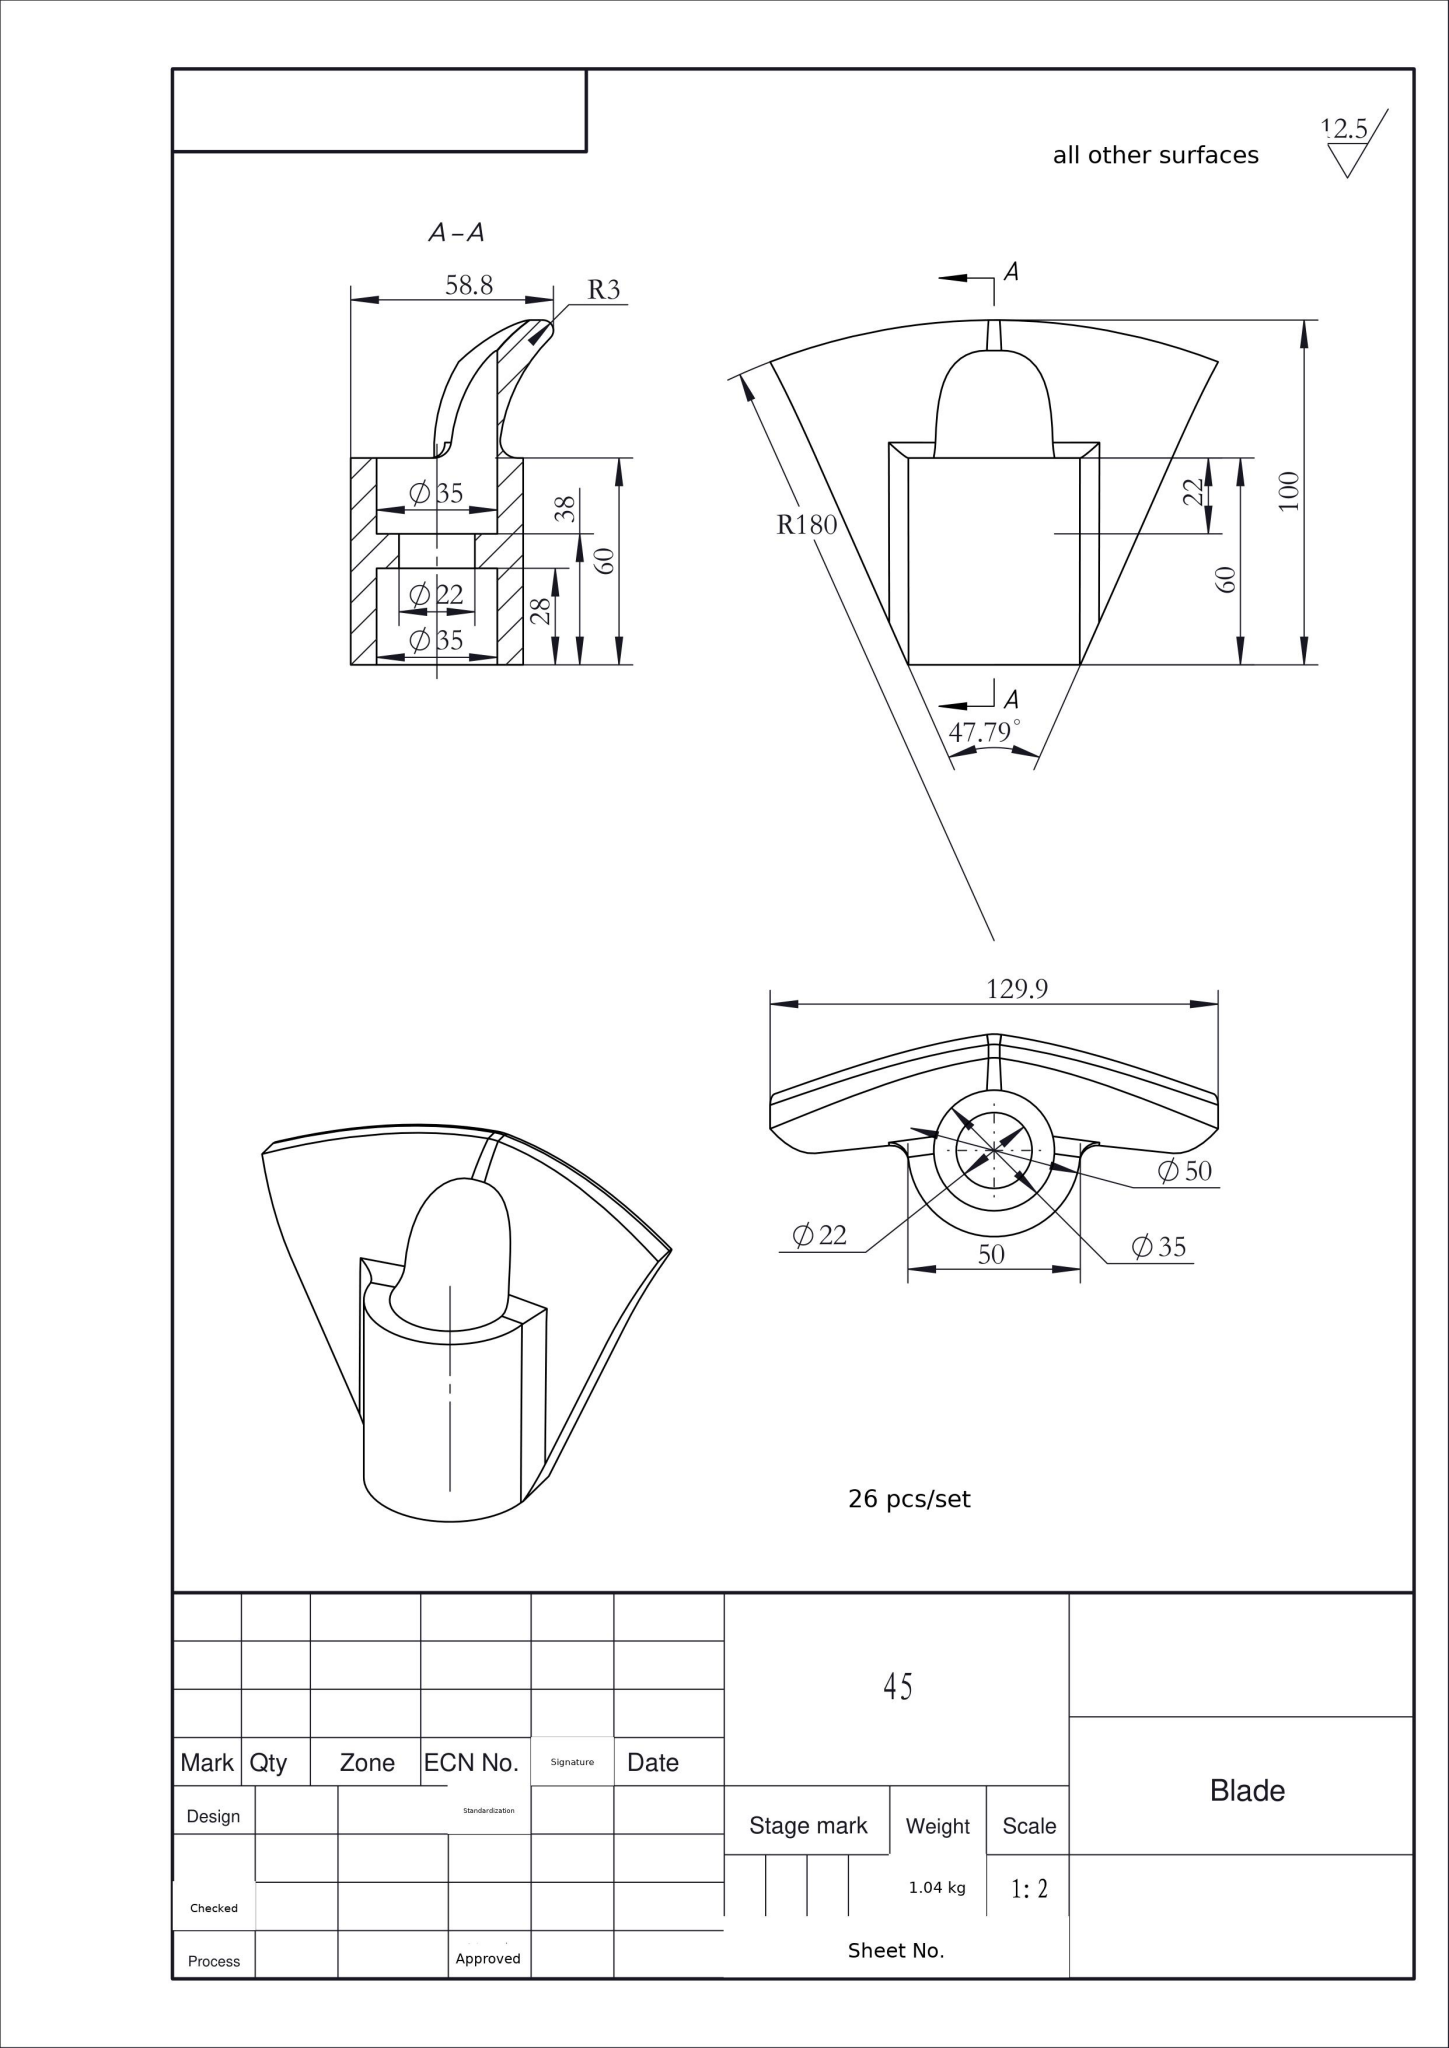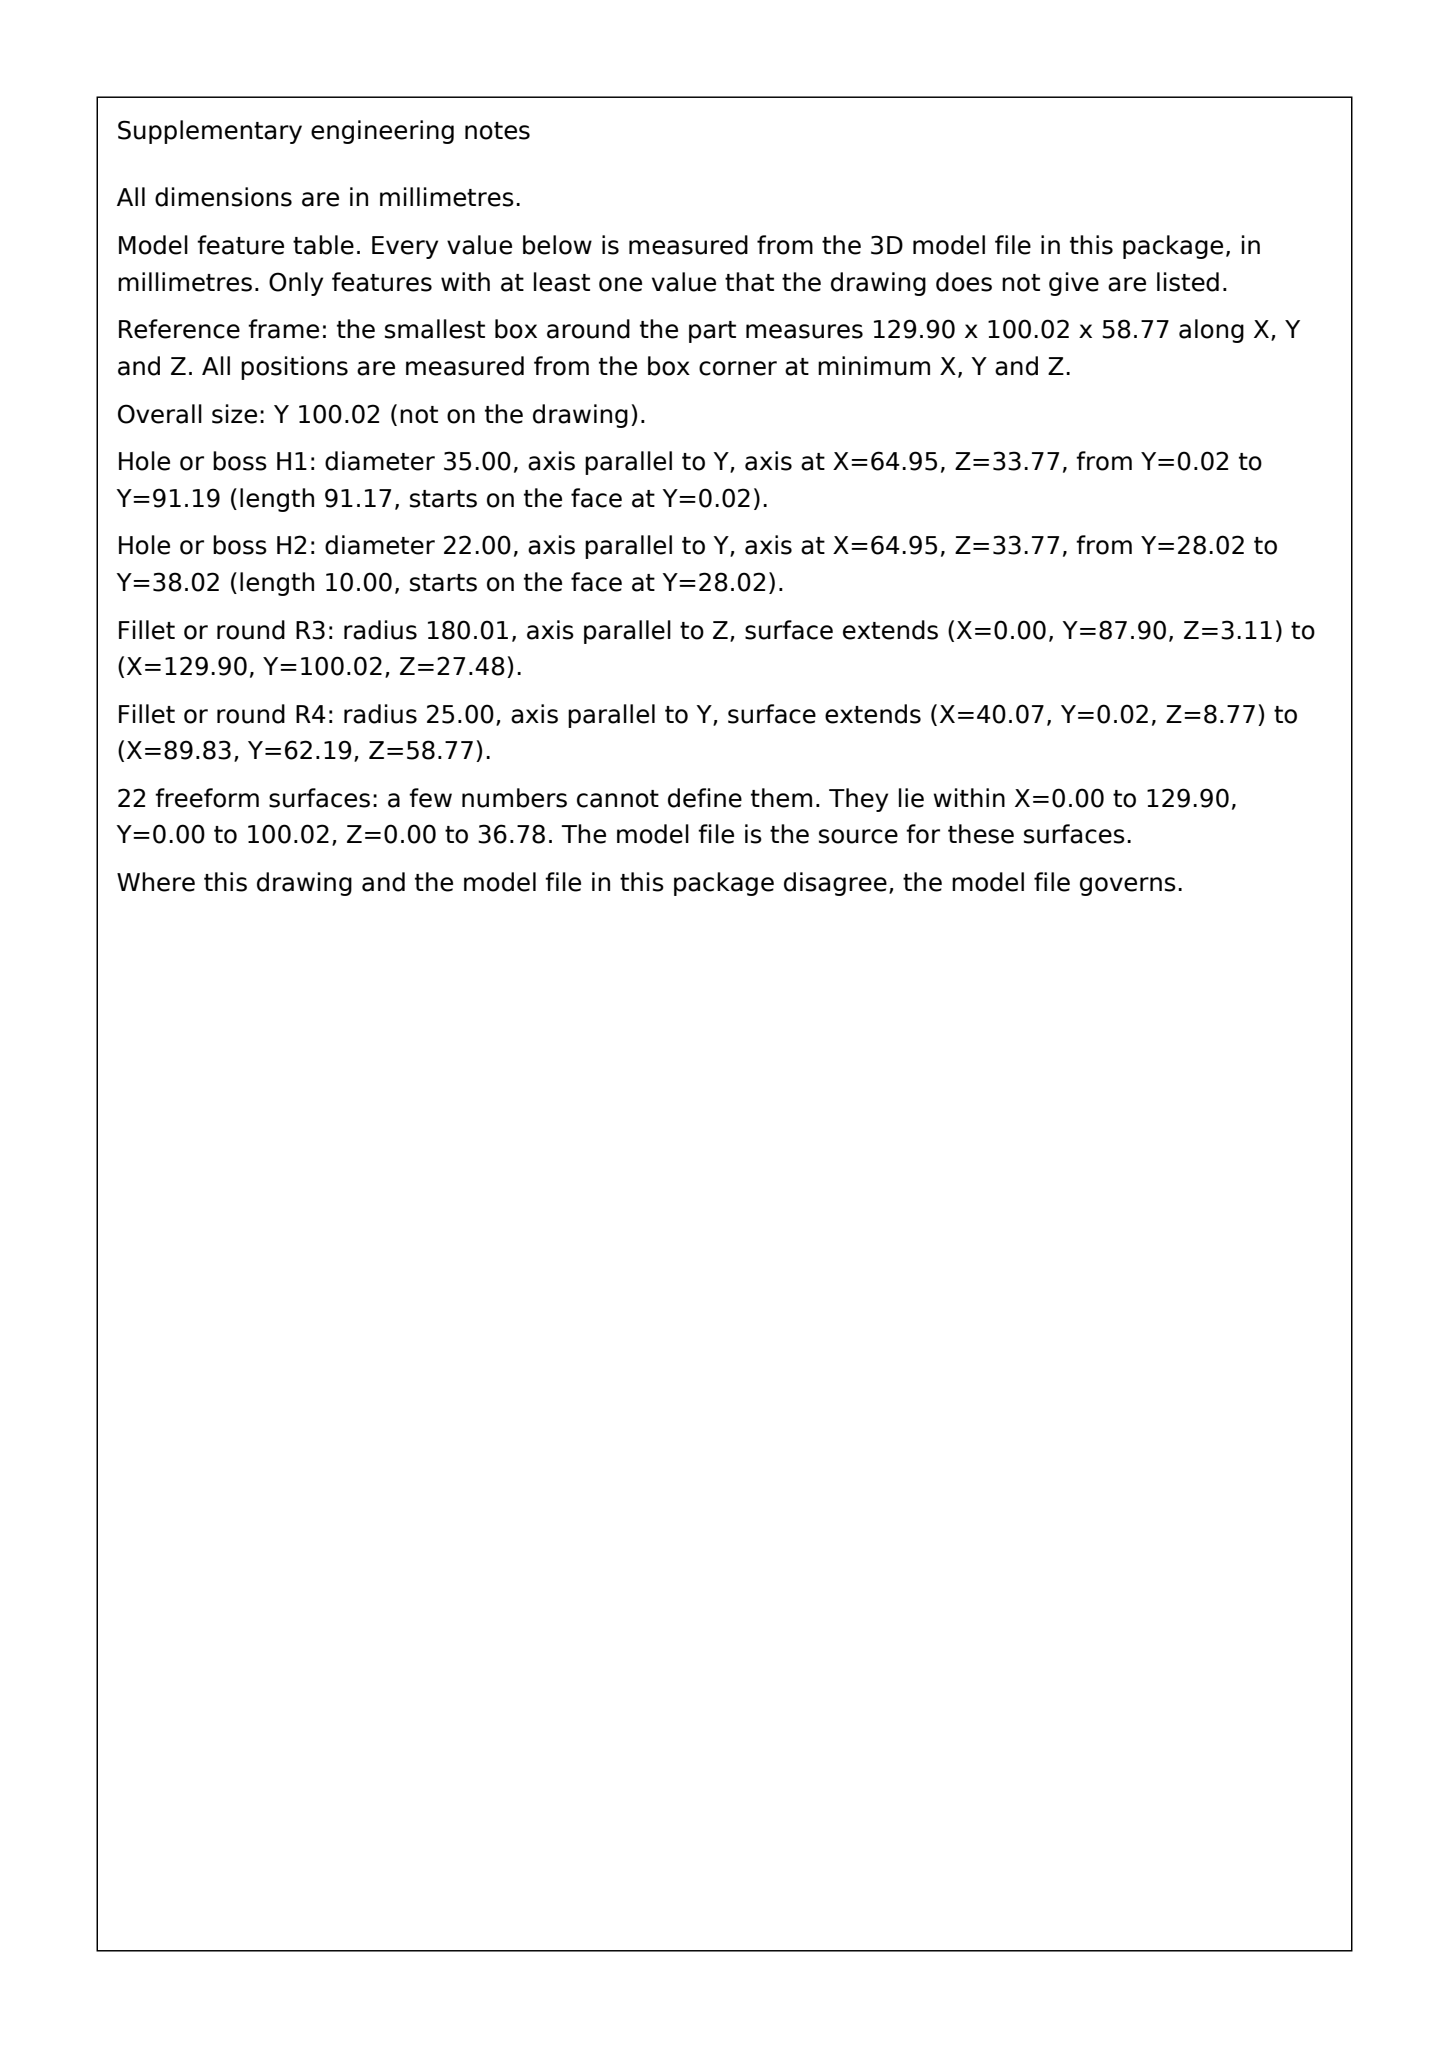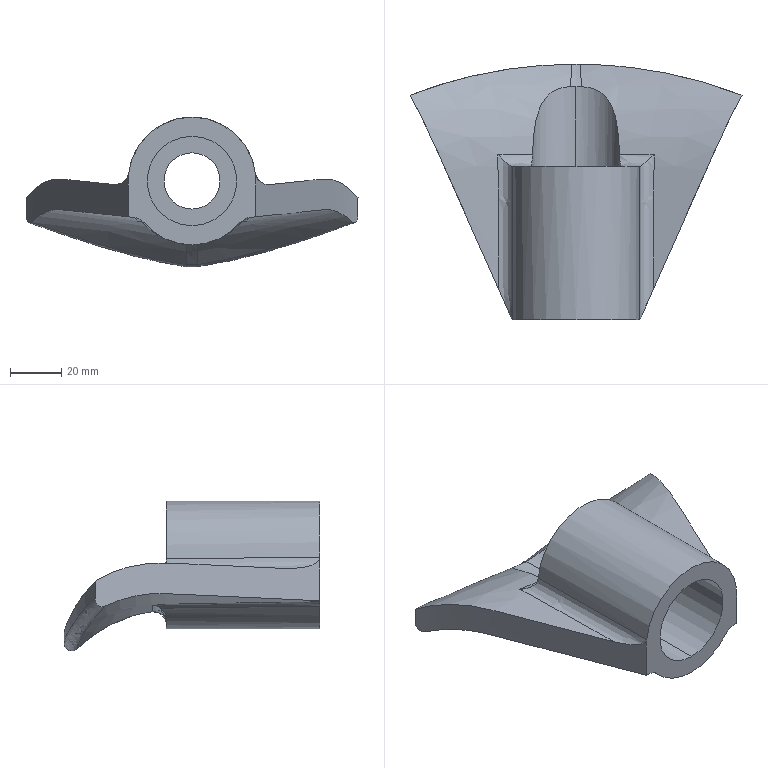Part | SolidWorks | mm | material 45 | 1 solid | 39 faces | box 129.9 x 100.02 x 58.77 mm | volume 133091 mm3 | spline 22 | cylinder 11 | plane 6 | commonest cylinder face diameters 35 x4 50 x3 22 x2 360.015 x2